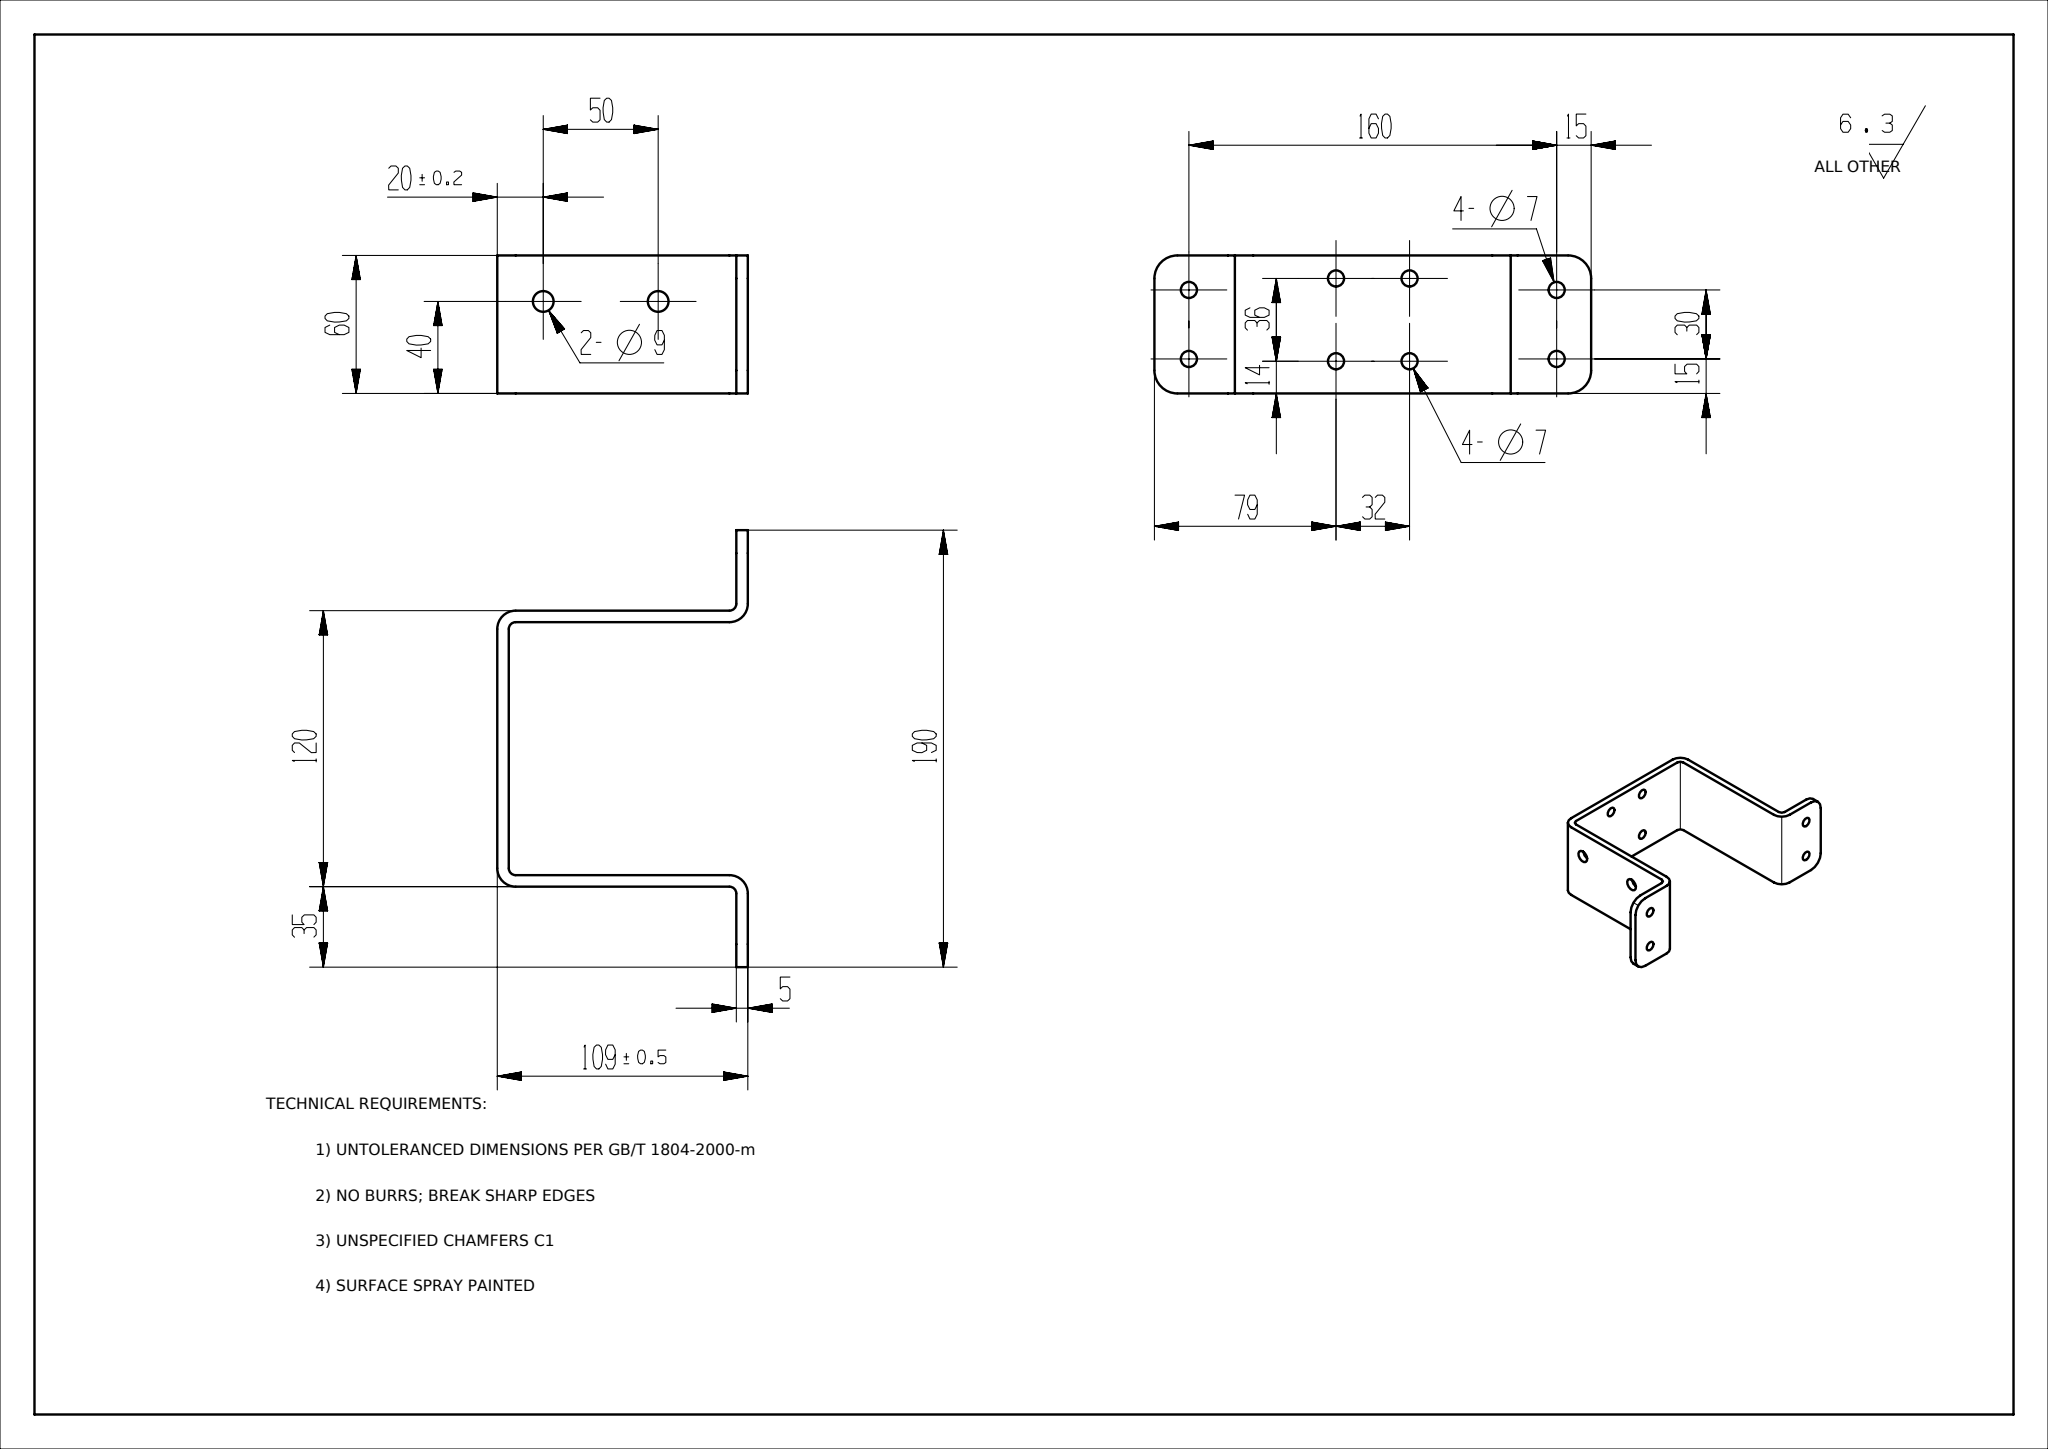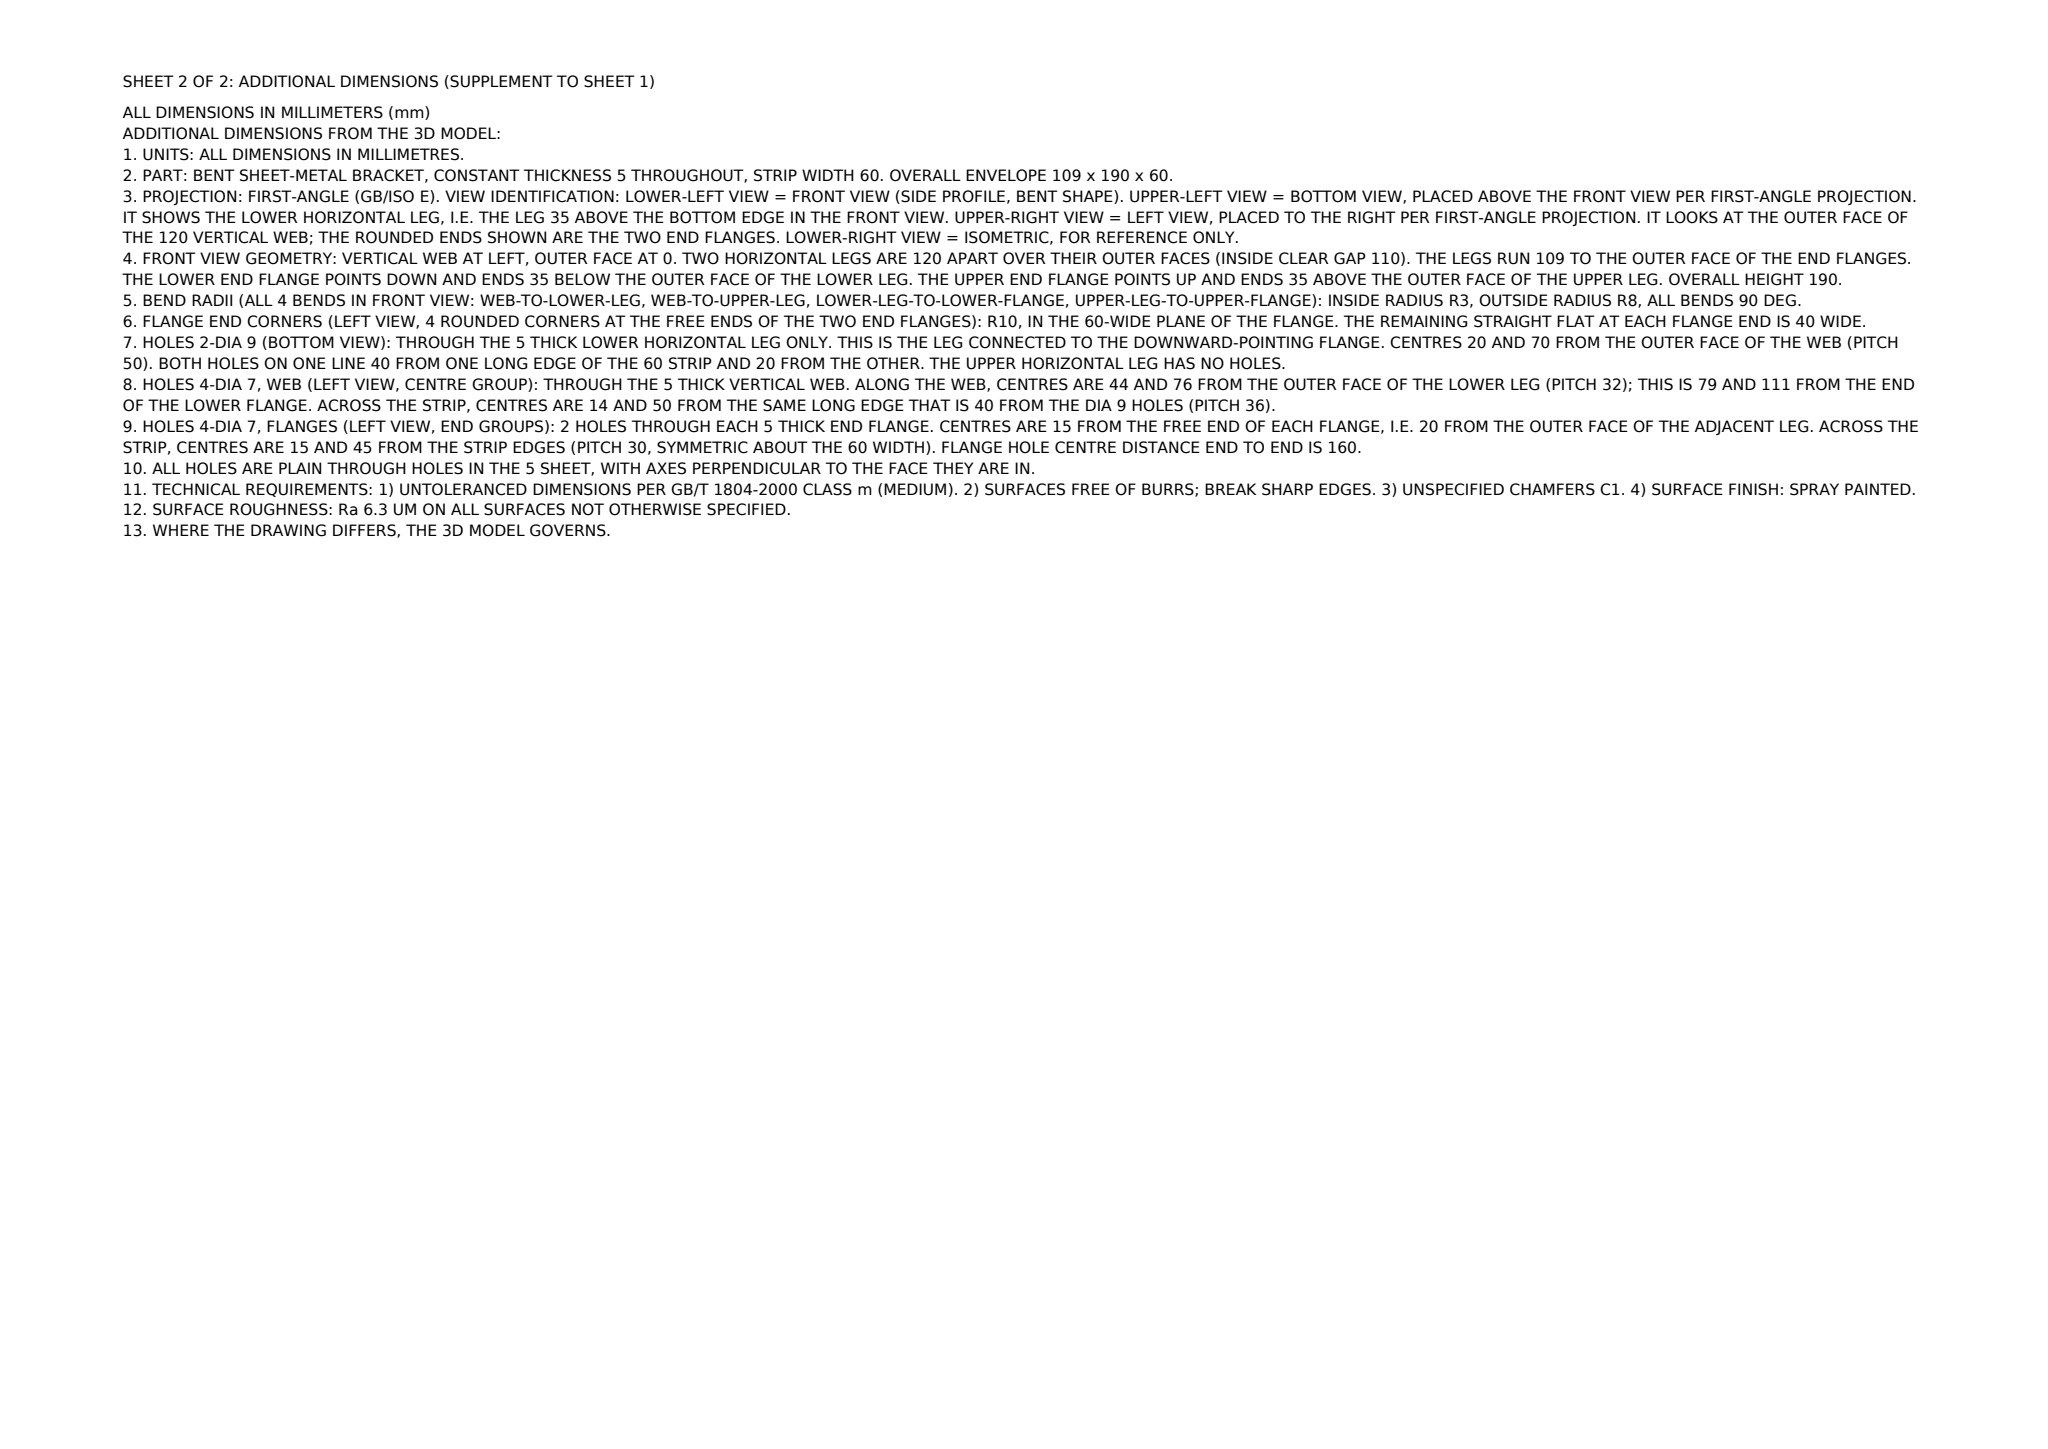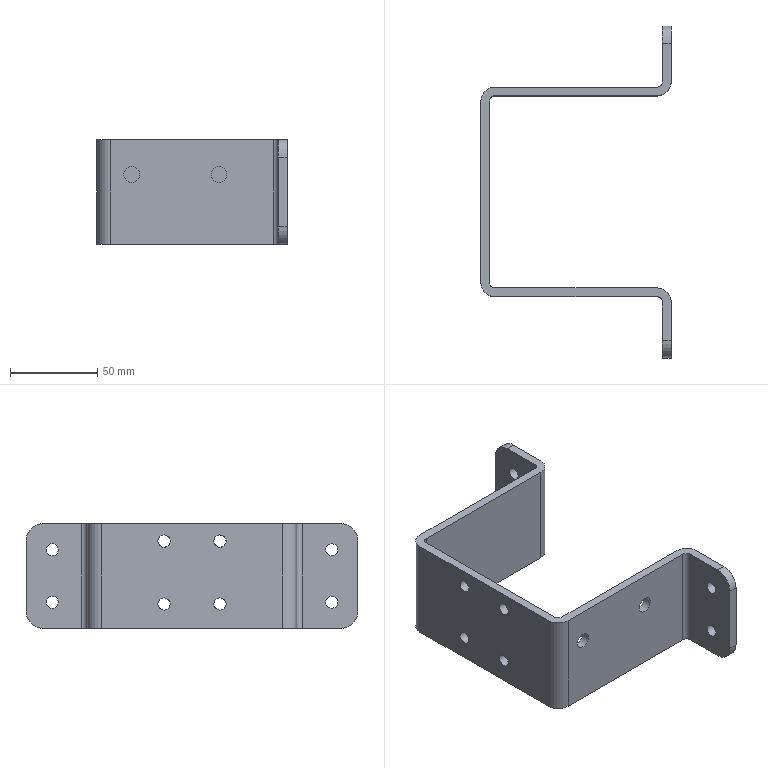Part | NX | mm | 1 solid | 36 faces | box 109 x 190 x 60 mm | volume 113962 mm3 | cylinder 22 | plane 14 | commonest cylinder face diameters 7 x8 6 x4 16 x4 20 x4 9 x2